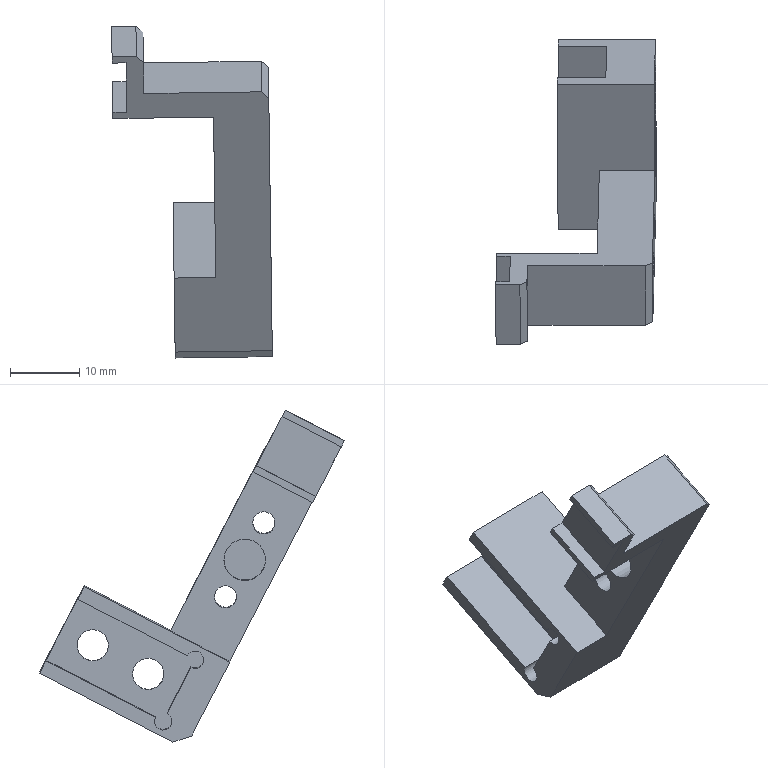Component | SolidWorks | 2018SOLIDWORKS1400000013-1 | 1 solid | 43 faces | box 23.16 x 43.92 x 47.84 mm | volume 5349 mm3 | plane 27 | cylinder 16 | commonest cylinder face diameters 8 x4 4.5 x4 6 x2 3.21 x2 3.2 x2 2.5 x2 | material 45 Steel
build123d program:
from build123d import *

# Parameters (mm, degrees)
SKETCH1_W                                       = 23.6
SKETCH1_H                                       = 14
BOSS_EXTRUDE1_DEPTH                             = 14
M4_HEX_SOCKET_HEAD_CAP_SCREW_CBORE1_D           = 4.5
M4_HEX_SOCKET_HEAD_CAP_SCREW_CBORE1_CBORE_D     = 8
M4_HEX_SOCKET_HEAD_CAP_SCREW_CBORE1_CBORE_DEPTH = 4.4
SKETCH45_W                                      = 19
SKETCH45_H                                      = 10
CUT_EXTRUDE24_DEPTH                             = 7
SKETCH46_R                                      = 1.25
CUT_EXTRUDE25_DEPTH                             = 7
SKETCH47_W                                      = 9.6
SKETCH47_H                                      = 8
BOSS_EXTRUDE2_DEPTH                             = 36
SKETCH48_W                                      = 9.6
SKETCH48_H                                      = 10
BOSS_EXTRUDE3_DEPTH                             = 14.5
SKETCH49_W                                      = 9.6
SKETCH49_H                                      = 8
CUT_EXTRUDE26_DEPTH                             = 2
CHAMFER1_SIZE                                   = 2
SKETCH50_R                                      = 1.6
SKETCH50_R_2                                    = 1.605
CUT_EXTRUDE27_DEPTH                             = 12
SKETCH51_R                                      = 3
CUT_EXTRUDE28_DEPTH                             = 6
SKETCH52_W                                      = 18
SKETCH52_H                                      = 20.853
CUT_EXTRUDE29_DEPTH                             = 15
CHAMFER2_SIZE                                   = 1
CHAMFER3_SIZE                                   = 2


with BuildPart() as part:
    # Sketch1 → Boss-Extrude1 (new body)
    with BuildSketch(Plane.XY):
        Rectangle(SKETCH1_W, SKETCH1_H)
    extrude(amount=BOSS_EXTRUDE1_DEPTH)

    # M4 Hex Socket Head Cap Screw CBORE1 (through all)
    with Locations(Plane.XY.offset(14)):
        with Locations((-6.8, 0), (2.2, 0)):
            CounterBoreHole(M4_HEX_SOCKET_HEAD_CAP_SCREW_CBORE1_D / 2, M4_HEX_SOCKET_HEAD_CAP_SCREW_CBORE1_CBORE_D / 2, M4_HEX_SOCKET_HEAD_CAP_SCREW_CBORE1_CBORE_DEPTH)

    # Sketch45 → Cut-Extrude24 (cut)
    with BuildSketch(Plane(origin=(0, 0, 0), x_dir=(-1, 0, 0), z_dir=(0, 0, -1))):
        with Locations((2.3, 0)):
            Rectangle(SKETCH45_W, SKETCH45_H)
    extrude(amount=-CUT_EXTRUDE24_DEPTH, mode=Mode.SUBTRACT)

    # Sketch46 → Cut-Extrude25 (cut)
    with BuildSketch(Plane(origin=(0, 0, 0), x_dir=(-1, 0, 0), z_dir=(0, 0, -1))):
        with Locations((-7.2, 5)):
            Circle(SKETCH46_R)
        with Locations((-7.2, -5)):
            Circle(SKETCH46_R)
    extrude(amount=-CUT_EXTRUDE25_DEPTH, mode=Mode.SUBTRACT)

    # Sketch47 → Boss-Extrude2 (add)
    with BuildSketch(Plane.XZ.offset(7)):
        with Locations((7, 10)):
            Rectangle(SKETCH47_W, SKETCH47_H)
    extrude(amount=BOSS_EXTRUDE2_DEPTH)

    # Sketch48 → Boss-Extrude3 (add)
    with BuildSketch(Plane(origin=(0, 0, 6), x_dir=(-1, 0, 0), z_dir=(0, 0, -1))):
        with Locations((-7, -38)):
            Rectangle(SKETCH48_W, SKETCH48_H)
    extrude(amount=BOSS_EXTRUDE3_DEPTH)

    # Sketch49 → Cut-Extrude26 (cut)
    with BuildSketch(Plane(origin=(0, 0, -8.5), x_dir=(-1, 0, 0), z_dir=(0, 0, -1))):
        with Locations((-7, -38)):
            Rectangle(SKETCH49_W, SKETCH49_H)
    extrude(amount=-CUT_EXTRUDE26_DEPTH, mode=Mode.SUBTRACT)

    # Chamfer1
    chamfer1_edges = [part.edges().sort_by_distance(p)[0] for p in [
        (7, -43, 14),
    ]]
    chamfer(chamfer1_edges, length=CHAMFER1_SIZE)

    # Sketch50 → Cut-Extrude27 (cut)
    with BuildSketch(Plane(origin=(0, 0, 6), x_dir=(-1, 0, 0), z_dir=(0, 0, -1))):
        with Locations((-7, -15)):
            Circle(SKETCH50_R)
        with Locations((-7, -27)):
            Circle(SKETCH50_R_2)
    extrude(amount=-CUT_EXTRUDE27_DEPTH, mode=Mode.SUBTRACT)

    # Sketch51 → Cut-Extrude28 (cut)
    with BuildSketch(Plane(origin=(0, 0, 6), x_dir=(-1, 0, 0), z_dir=(0, 0, -1))):
        with Locations((-7, -21)):
            Circle(SKETCH51_R)
    extrude(amount=-CUT_EXTRUDE28_DEPTH, mode=Mode.SUBTRACT)

    # Sketch52 → Cut-Extrude29 (cut)
    with BuildSketch(Plane.ZY.offset(-2.2)):
        with Locations((5, -47.427)):
            Rectangle(SKETCH52_W, SKETCH52_H)
    extrude(amount=-CUT_EXTRUDE29_DEPTH, mode=Mode.SUBTRACT)

    # Chamfer2
    chamfer2_edges = [part.edges().sort_by_distance(p)[0] for p in [
        (7, -43, -4),
        (7, -37, 14),
    ]]
    chamfer(chamfer2_edges, length=CHAMFER2_SIZE)

    # Chamfer3
    chamfer3_edges = [part.edges().sort_by_distance(p)[0] for p in [
        (11.8, 7, 7),
    ]]
    chamfer(chamfer3_edges, length=CHAMFER3_SIZE)


solid = part.part

# Placed as in the assembly
solid = solid.moved(Location((111.072, -82.786, 161.815), (0, 89.207, -62.677)))